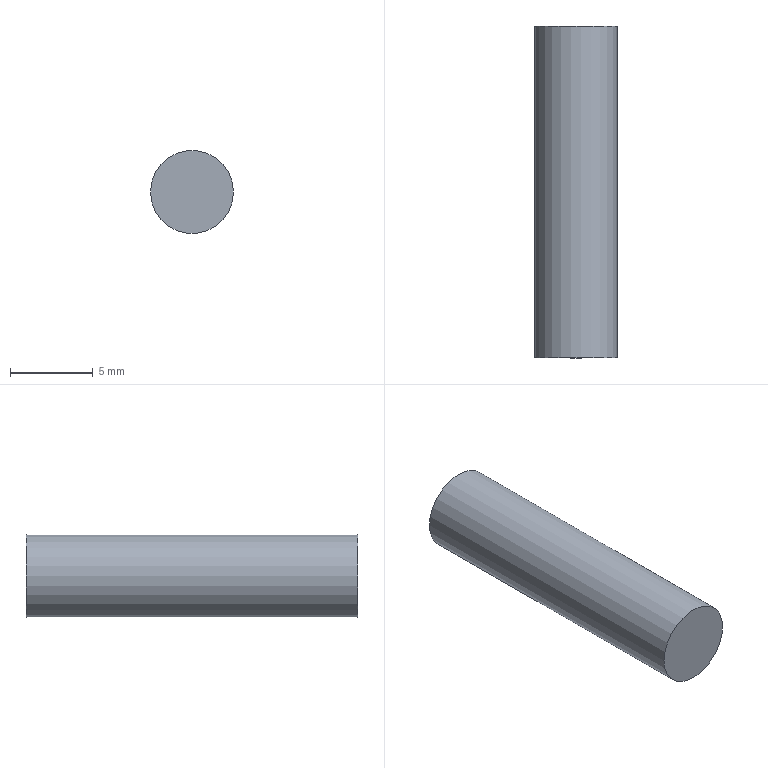Component | NX | DOWEL_PIN_5_20_2 | 1 solid | 3 faces | box 5 x 20 x 5 mm | volume 393 mm3 | plane 2 | cylinder 1 | commonest cylinder face diameters 5 x1
STEP:
#1=CARTESIAN_POINT('',(0.,0.,0.));
#2=DIRECTION('',(0.,0.,1.));
#3=DIRECTION('',(1.,0.,0.));
#4=AXIS2_PLACEMENT_3D('',#1,#2,#3);
#5=CARTESIAN_POINT('',(-24.5,-6.,19.));
#6=VERTEX_POINT('',#5);
#7=CARTESIAN_POINT('',(-27.,-6.,19.));
#8=DIRECTION('',(0.,1.,0.));
#9=DIRECTION('',(1.,0.,0.));
#10=AXIS2_PLACEMENT_3D('',#7,#8,#9);
#11=CIRCLE('',#10,2.5);
#12=CARTESIAN_POINT('',(-27.,-6.,19.));
#13=DIRECTION('',(0.,-1.,0.));
#14=DIRECTION('',(-1.,0.,0.));
#15=AXIS2_PLACEMENT_3D('',#12,#13,#14);
#16=CYLINDRICAL_SURFACE('',#15,2.5);
#17=CARTESIAN_POINT('',(9.425,0.));
#18=DIRECTION('',(-1.,0.));
#19=VECTOR('',#18,1.);
#20=LINE('',#17,#19);
#21=(GEOMETRIC_REPRESENTATION_CONTEXT(2)PARAMETRIC_REPRESENTATION_CONTEXT()REPRESENTATION_CONTEXT('',''));
#22=DEFINITIONAL_REPRESENTATION('',(#20),#21);
#23=PCURVE('',#16,#22);
#24=CARTESIAN_POINT('',(-27.,-6.,19.));
#25=DIRECTION('',(0.,1.,0.));
#26=DIRECTION('',(1.,0.,0.));
#27=AXIS2_PLACEMENT_3D('',#24,#25,#26);
#28=PLANE('',#27);
#29=CARTESIAN_POINT('',(0.,0.));
#30=DIRECTION('',(1.,0.));
#31=AXIS2_PLACEMENT_2D('',#29,#30);
#32=CIRCLE('',#31,2.5);
#33=(GEOMETRIC_REPRESENTATION_CONTEXT(2)PARAMETRIC_REPRESENTATION_CONTEXT()REPRESENTATION_CONTEXT('',''));
#34=DEFINITIONAL_REPRESENTATION('',(#32),#33);
#35=PCURVE('',#28,#34);
#36=SURFACE_CURVE('',#11,(#23,#35),.PCURVE_S1.);
#37=EDGE_CURVE('',#6,#6,#36,.T.);
#38=ORIENTED_EDGE('',*,*,#37,.F.);
#39=CARTESIAN_POINT('',(-24.5,-26.,19.));
#40=VERTEX_POINT('',#39);
#41=CARTESIAN_POINT('',(-24.5,-6.,19.));
#42=CARTESIAN_POINT('',(-24.5,-26.,19.));
#43=B_SPLINE_CURVE_WITH_KNOTS('',1,(#41,#42),.UNSPECIFIED.,.F.,.F.,(2,2),(0.,20.),.PIECEWISE_BEZIER_KNOTS.);
#44=CARTESIAN_POINT('',(9.425,0.));
#45=DIRECTION('',(0.,1.));
#46=VECTOR('',#45,1.);
#47=LINE('',#44,#46);
#48=(GEOMETRIC_REPRESENTATION_CONTEXT(2)PARAMETRIC_REPRESENTATION_CONTEXT()REPRESENTATION_CONTEXT('',''));
#49=DEFINITIONAL_REPRESENTATION('',(#47),#48);
#50=PCURVE('',#16,#49);
#51=CARTESIAN_POINT('',(3.142,0.));
#52=DIRECTION('',(0.,1.));
#53=VECTOR('',#52,1.);
#54=LINE('',#51,#53);
#55=(GEOMETRIC_REPRESENTATION_CONTEXT(2)PARAMETRIC_REPRESENTATION_CONTEXT()REPRESENTATION_CONTEXT('',''));
#56=DEFINITIONAL_REPRESENTATION('',(#54),#55);
#57=PCURVE('',#16,#56);
#58=SEAM_CURVE('',#43,(#50,#57),.PCURVE_S1.);
#59=EDGE_CURVE('',#6,#40,#58,.T.);
#60=ORIENTED_EDGE('',*,*,#59,.T.);
#61=CARTESIAN_POINT('',(-27.,-26.,19.));
#62=DIRECTION('',(0.,1.,0.));
#63=DIRECTION('',(1.,0.,0.));
#64=AXIS2_PLACEMENT_3D('',#61,#62,#63);
#65=CIRCLE('',#64,2.5);
#66=CARTESIAN_POINT('',(9.425,20.));
#67=DIRECTION('',(-1.,0.));
#68=VECTOR('',#67,1.);
#69=LINE('',#66,#68);
#70=(GEOMETRIC_REPRESENTATION_CONTEXT(2)PARAMETRIC_REPRESENTATION_CONTEXT()REPRESENTATION_CONTEXT('',''));
#71=DEFINITIONAL_REPRESENTATION('',(#69),#70);
#72=PCURVE('',#16,#71);
#73=CARTESIAN_POINT('',(-27.,-26.,19.));
#74=DIRECTION('',(0.,1.,0.));
#75=DIRECTION('',(1.,0.,0.));
#76=AXIS2_PLACEMENT_3D('',#73,#74,#75);
#77=PLANE('',#76);
#78=CARTESIAN_POINT('',(0.,0.));
#79=DIRECTION('',(1.,0.));
#80=AXIS2_PLACEMENT_2D('',#78,#79);
#81=CIRCLE('',#80,2.5);
#82=(GEOMETRIC_REPRESENTATION_CONTEXT(2)PARAMETRIC_REPRESENTATION_CONTEXT()REPRESENTATION_CONTEXT('',''));
#83=DEFINITIONAL_REPRESENTATION('',(#81),#82);
#84=PCURVE('',#77,#83);
#85=SURFACE_CURVE('',#65,(#72,#84),.PCURVE_S1.);
#86=EDGE_CURVE('',#40,#40,#85,.T.);
#87=ORIENTED_EDGE('',*,*,#86,.T.);
#88=ORIENTED_EDGE('',*,*,#59,.F.);
#89=EDGE_LOOP('',(#38,#60,#87,#88));
#90=FACE_BOUND('',#89,.T.);
#91=ADVANCED_FACE('',(#90),#16,.T.);
#92=ORIENTED_EDGE('',*,*,#37,.T.);
#93=EDGE_LOOP('',(#92));
#94=FACE_BOUND('',#93,.T.);
#95=ADVANCED_FACE('',(#94),#28,.T.);
#96=ORIENTED_EDGE('',*,*,#86,.F.);
#97=EDGE_LOOP('',(#96));
#98=FACE_BOUND('',#97,.T.);
#99=ADVANCED_FACE('',(#98),#77,.F.);
#100=CLOSED_SHELL('',(#91,#95,#99));
#101=MANIFOLD_SOLID_BREP('',#100);
#102=(LENGTH_UNIT()NAMED_UNIT(*)SI_UNIT(.MILLI.,.METRE.));
#103=UNCERTAINTY_MEASURE_WITH_UNIT(LENGTH_MEASURE(0.00001),#102,'','');
#104=(NAMED_UNIT(*)PLANE_ANGLE_UNIT()SI_UNIT($,.RADIAN.));
#105=(NAMED_UNIT(*)SI_UNIT($,.STERADIAN.)SOLID_ANGLE_UNIT());
#106=(GEOMETRIC_REPRESENTATION_CONTEXT(3)GLOBAL_UNCERTAINTY_ASSIGNED_CONTEXT((#103))GLOBAL_UNIT_ASSIGNED_CONTEXT((#102,#104,#105))REPRESENTATION_CONTEXT('',''));
#107=ADVANCED_BREP_SHAPE_REPRESENTATION('',(#4,#101),#106);